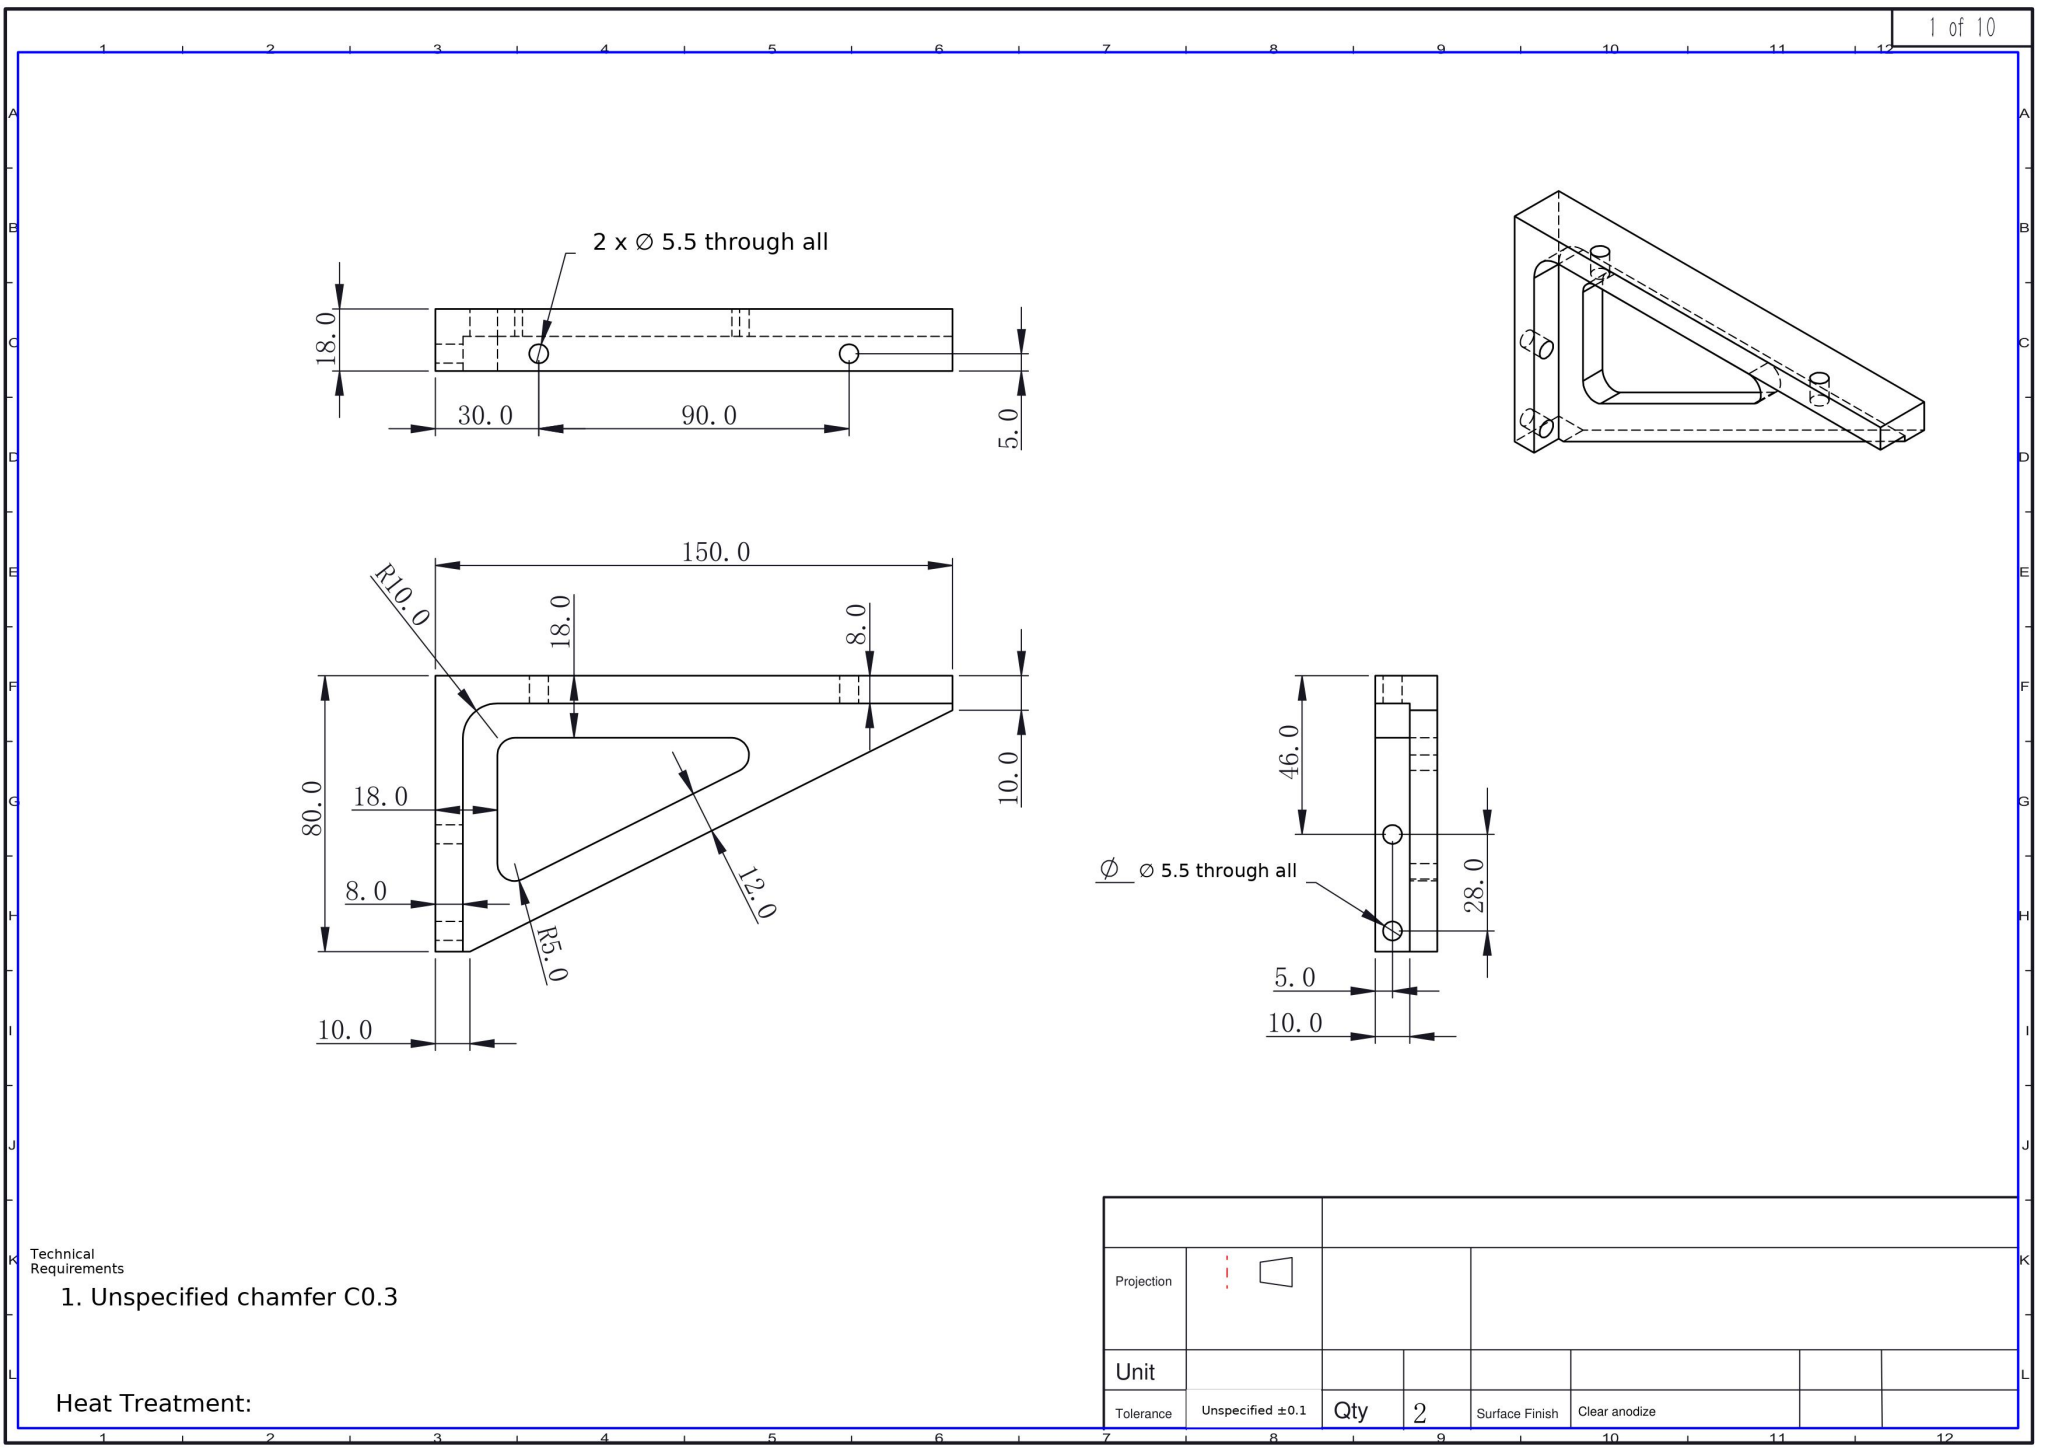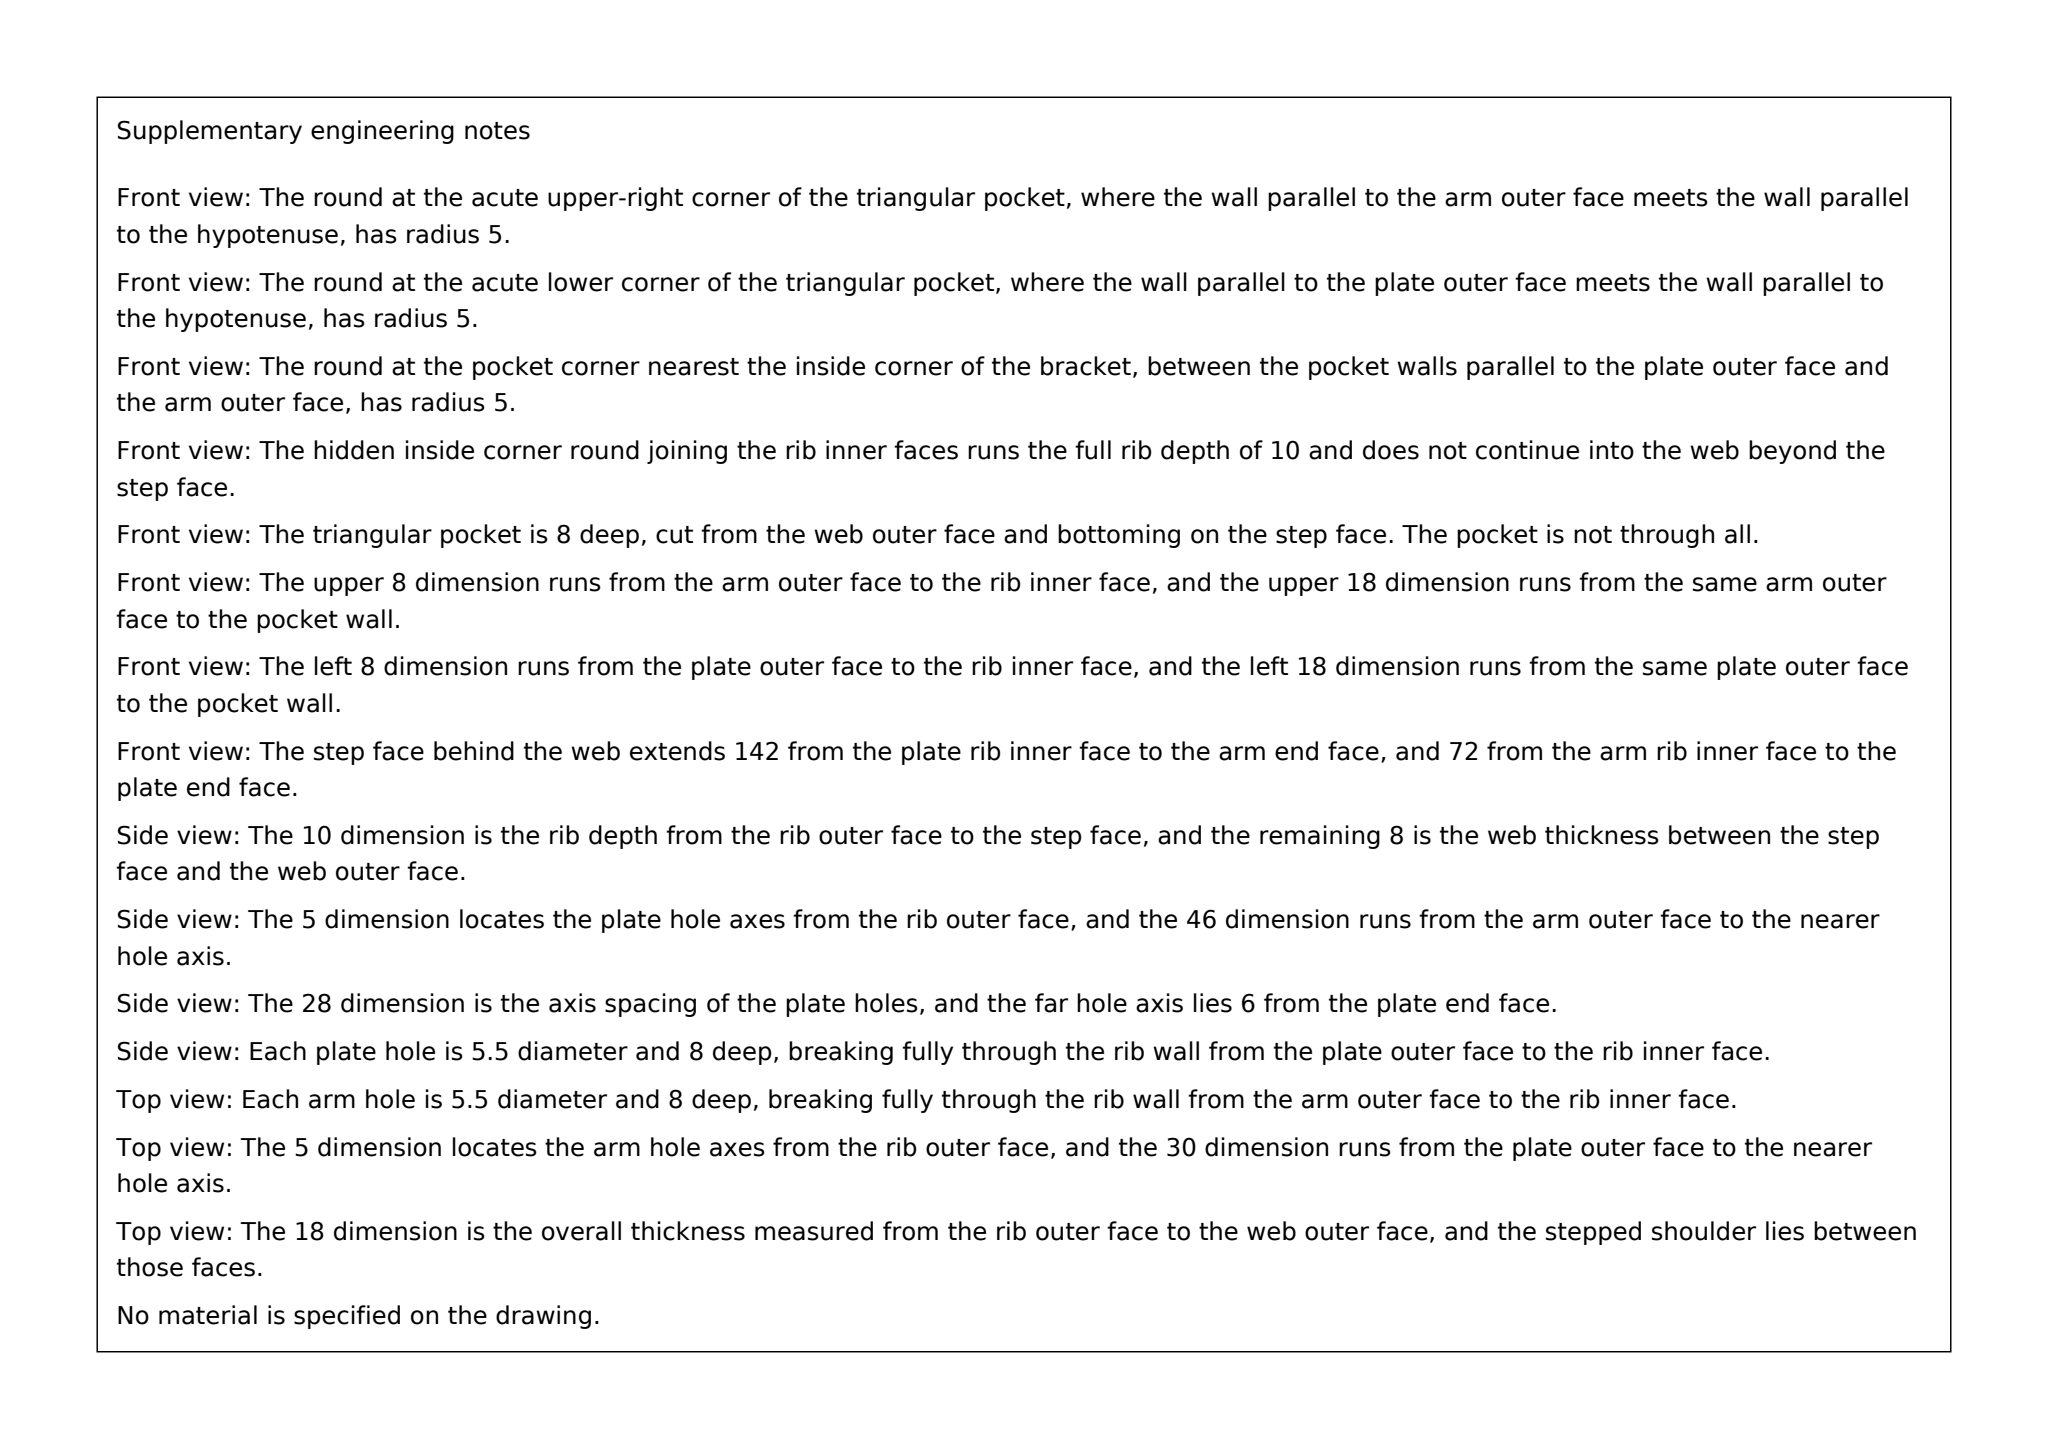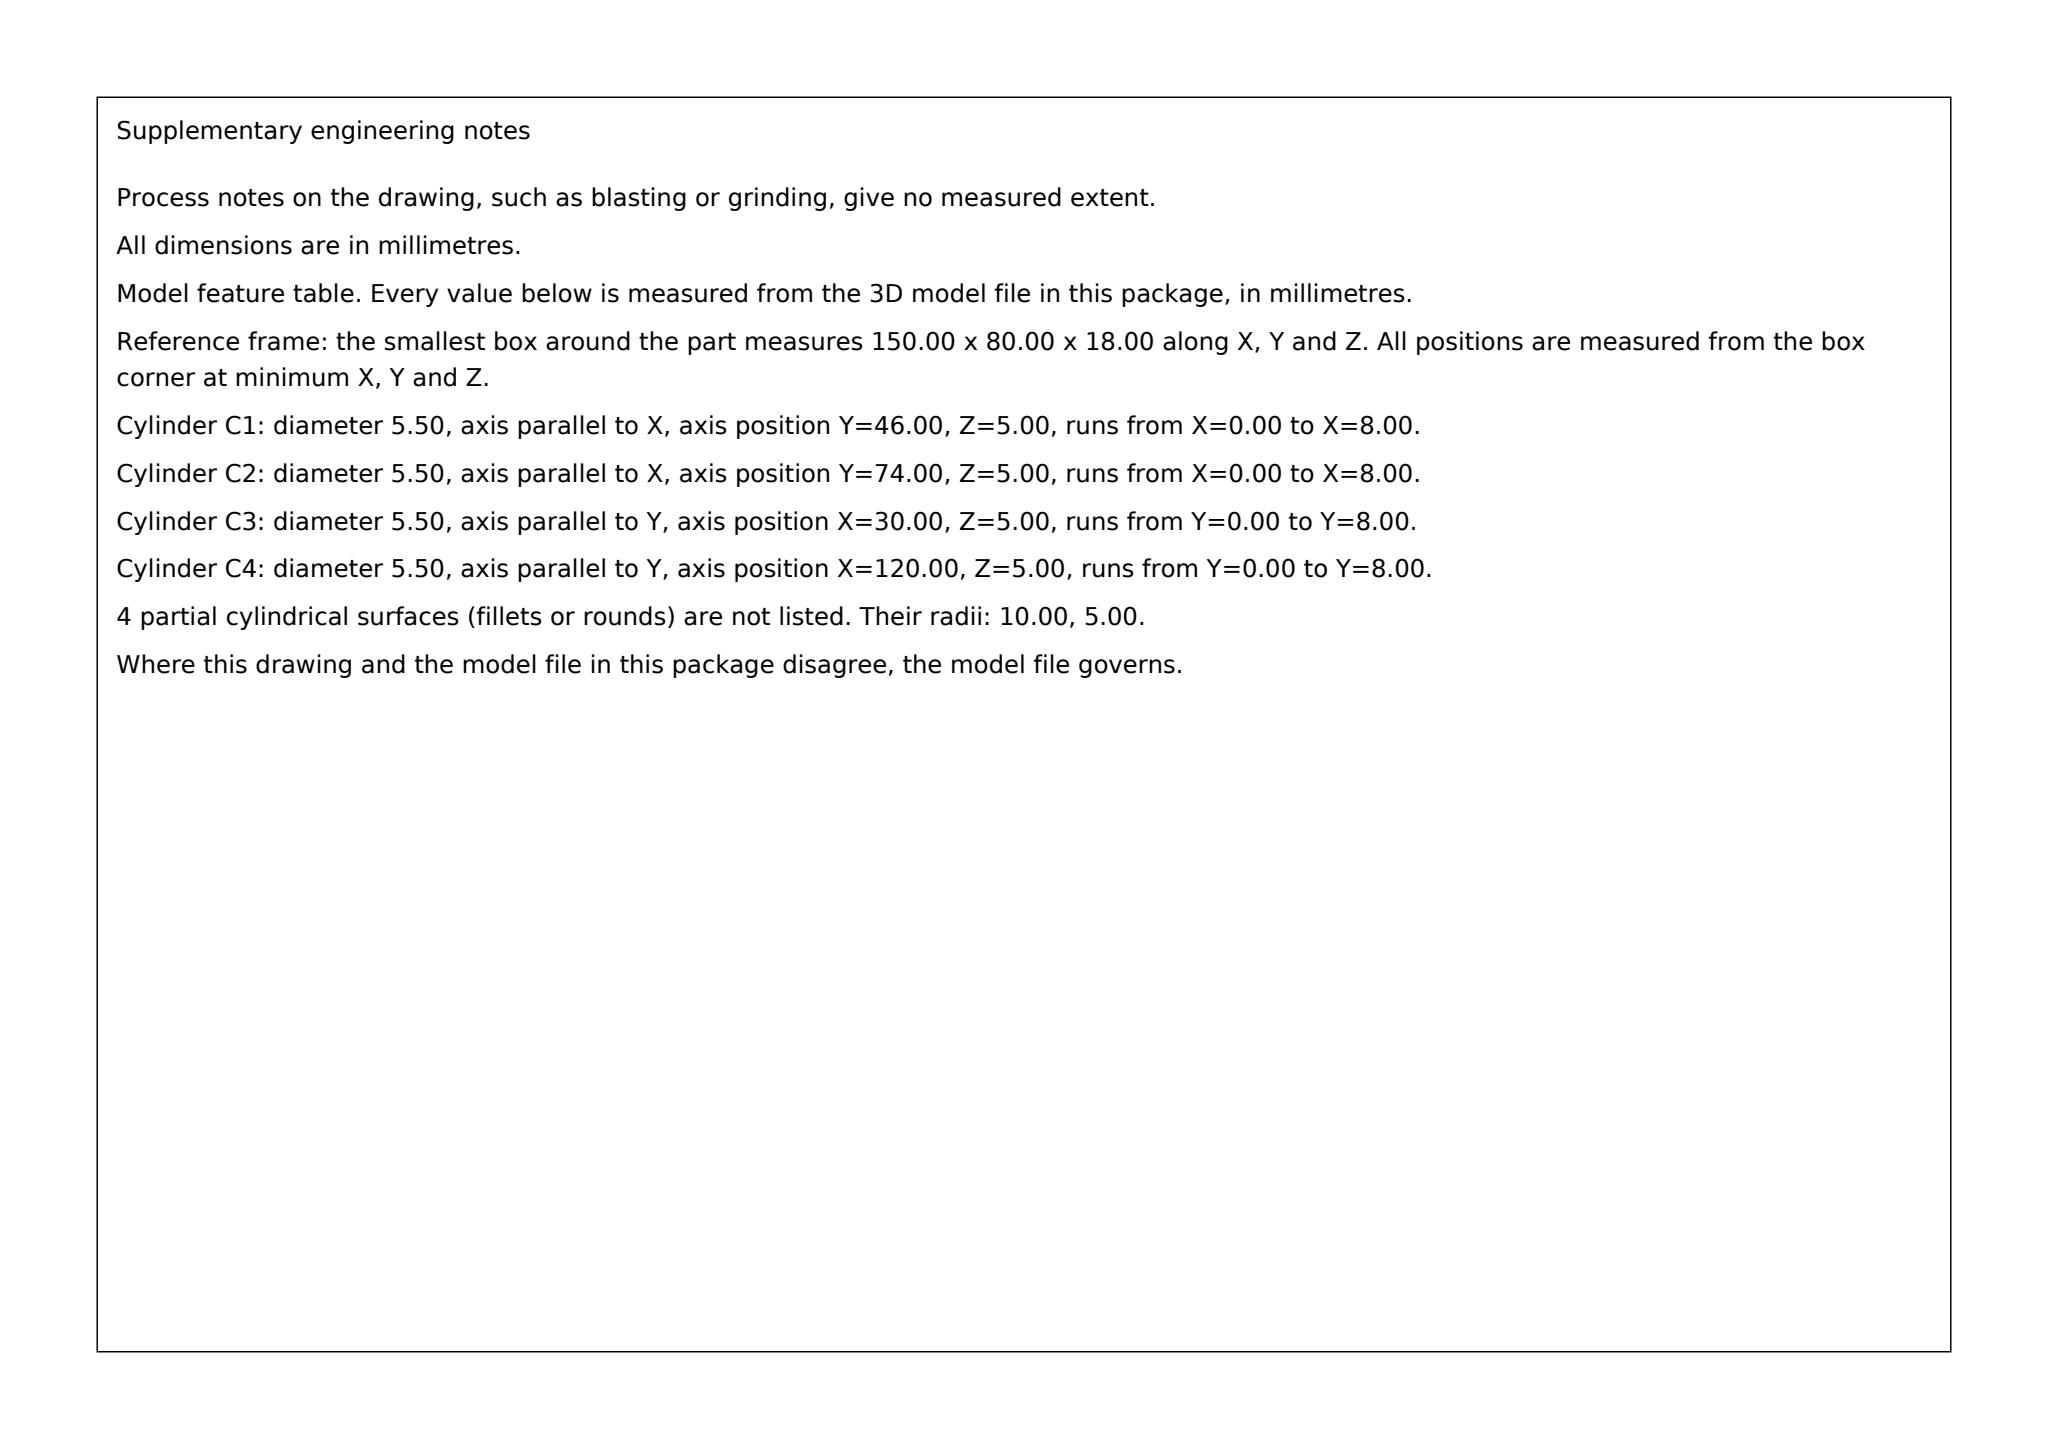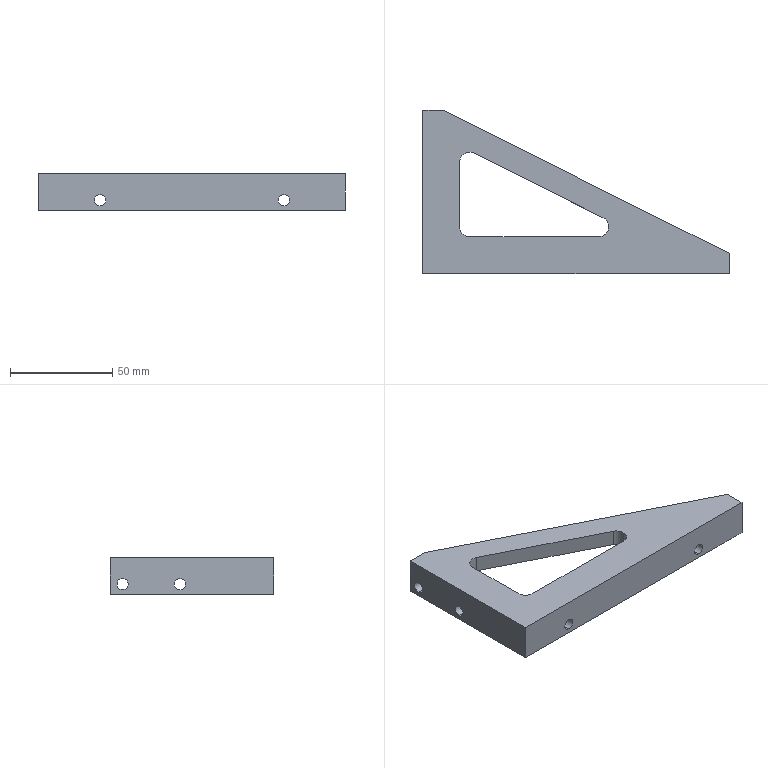Part | SolidWorks | mm | 1 solid | 25 faces | box 150 x 80 x 18 mm | volume 58855 mm3 | plane 13 | cylinder 12 | commonest cylinder face diameters 5.5 x8 10 x3 20 x1
Drawing notes:
SIDE VIEW: 2 X Ø5.5 THRU ALL, 28 APART, @ 46 & 74 FROM BASE | from the solid: cylinders dia 5.5 axis x at y=46.0 and y=74.0, z=5.0, len 8.0 (bbox Y=80)
build123d program:
from build123d import *

# Parameters (mm, degrees)
BOSS_EXTRUDE1_DEPTH   = 18
CUT_EXTRUDE2_DEPTH    = 10
CUT_EXTRUDE3_DEPTH    = 171.294
M5_CLEARANCE_HOLE_1_D = 5.5
M5_CLEARANCE_HOLE_2_D = 5.5


with BuildPart() as part:
    # Sketch1 → Boss-Extrude1 (new body)
    with BuildSketch(Plane.XY):
        Polygon((10, 80), (150, 10), (150, 0), (0, 0), (0, 80), align=None)
    extrude(amount=BOSS_EXTRUDE1_DEPTH)

    # Sketch10 → Cut-Extrude2 (cut)
    with BuildSketch(Plane(origin=(0, 0, 0), x_dir=(-1, 0, 0), z_dir=(0, 0, -1))):
        with BuildLine():
            Line((-8, 80), (-150, 80))
            Line((-150, 80), (-150, 8))
            Line((-150, 8), (-18, 8))
            ThreePointArc((-18, 8), (-10.929, 10.929), (-8, 18))
            Line((-8, 18), (-8, 80))
        make_face()
    extrude(amount=-CUT_EXTRUDE2_DEPTH, mode=Mode.SUBTRACT)

    # Sketch11 → Cut-Extrude3 (cut, through all)
    with BuildSketch(Plane(origin=(0, 0, 10), x_dir=(-1, 0, 0), z_dir=(0, 0, -1))):
        with BuildLine():
            Line((-18, 23), (-18, 54.493))
            ThreePointArc((-18, 54.493), (-20.371, 58.747), (-25.236, 58.966))
            Line((-25.236, 58.966), (-88.223, 27.472))
            ThreePointArc((-88.223, 27.472), (-90.853, 21.851), (-85.987, 18))
            Line((-85.987, 18), (-23, 18))
            ThreePointArc((-23, 18), (-19.464, 19.464), (-18, 23))
        make_face()
    extrude(amount=-CUT_EXTRUDE3_DEPTH, mode=Mode.SUBTRACT)

    # M5 Clearance Hole 1 (through all)
    with Locations(Plane(origin=(8, 0, 0), x_dir=(0, 0, -1), z_dir=(1, 0, 0))):
        with Locations((-5, 46), (-5, 74)):
            Hole(M5_CLEARANCE_HOLE_1_D / 2)

    # M5 Clearance Hole 2 (through all)
    with Locations(Plane(origin=(0, 8, 0), x_dir=(1, 0, 0), z_dir=(0, 1, 0))):
        with Locations((30, -5), (120, -5)):
            Hole(M5_CLEARANCE_HOLE_2_D / 2)


solid = part.part